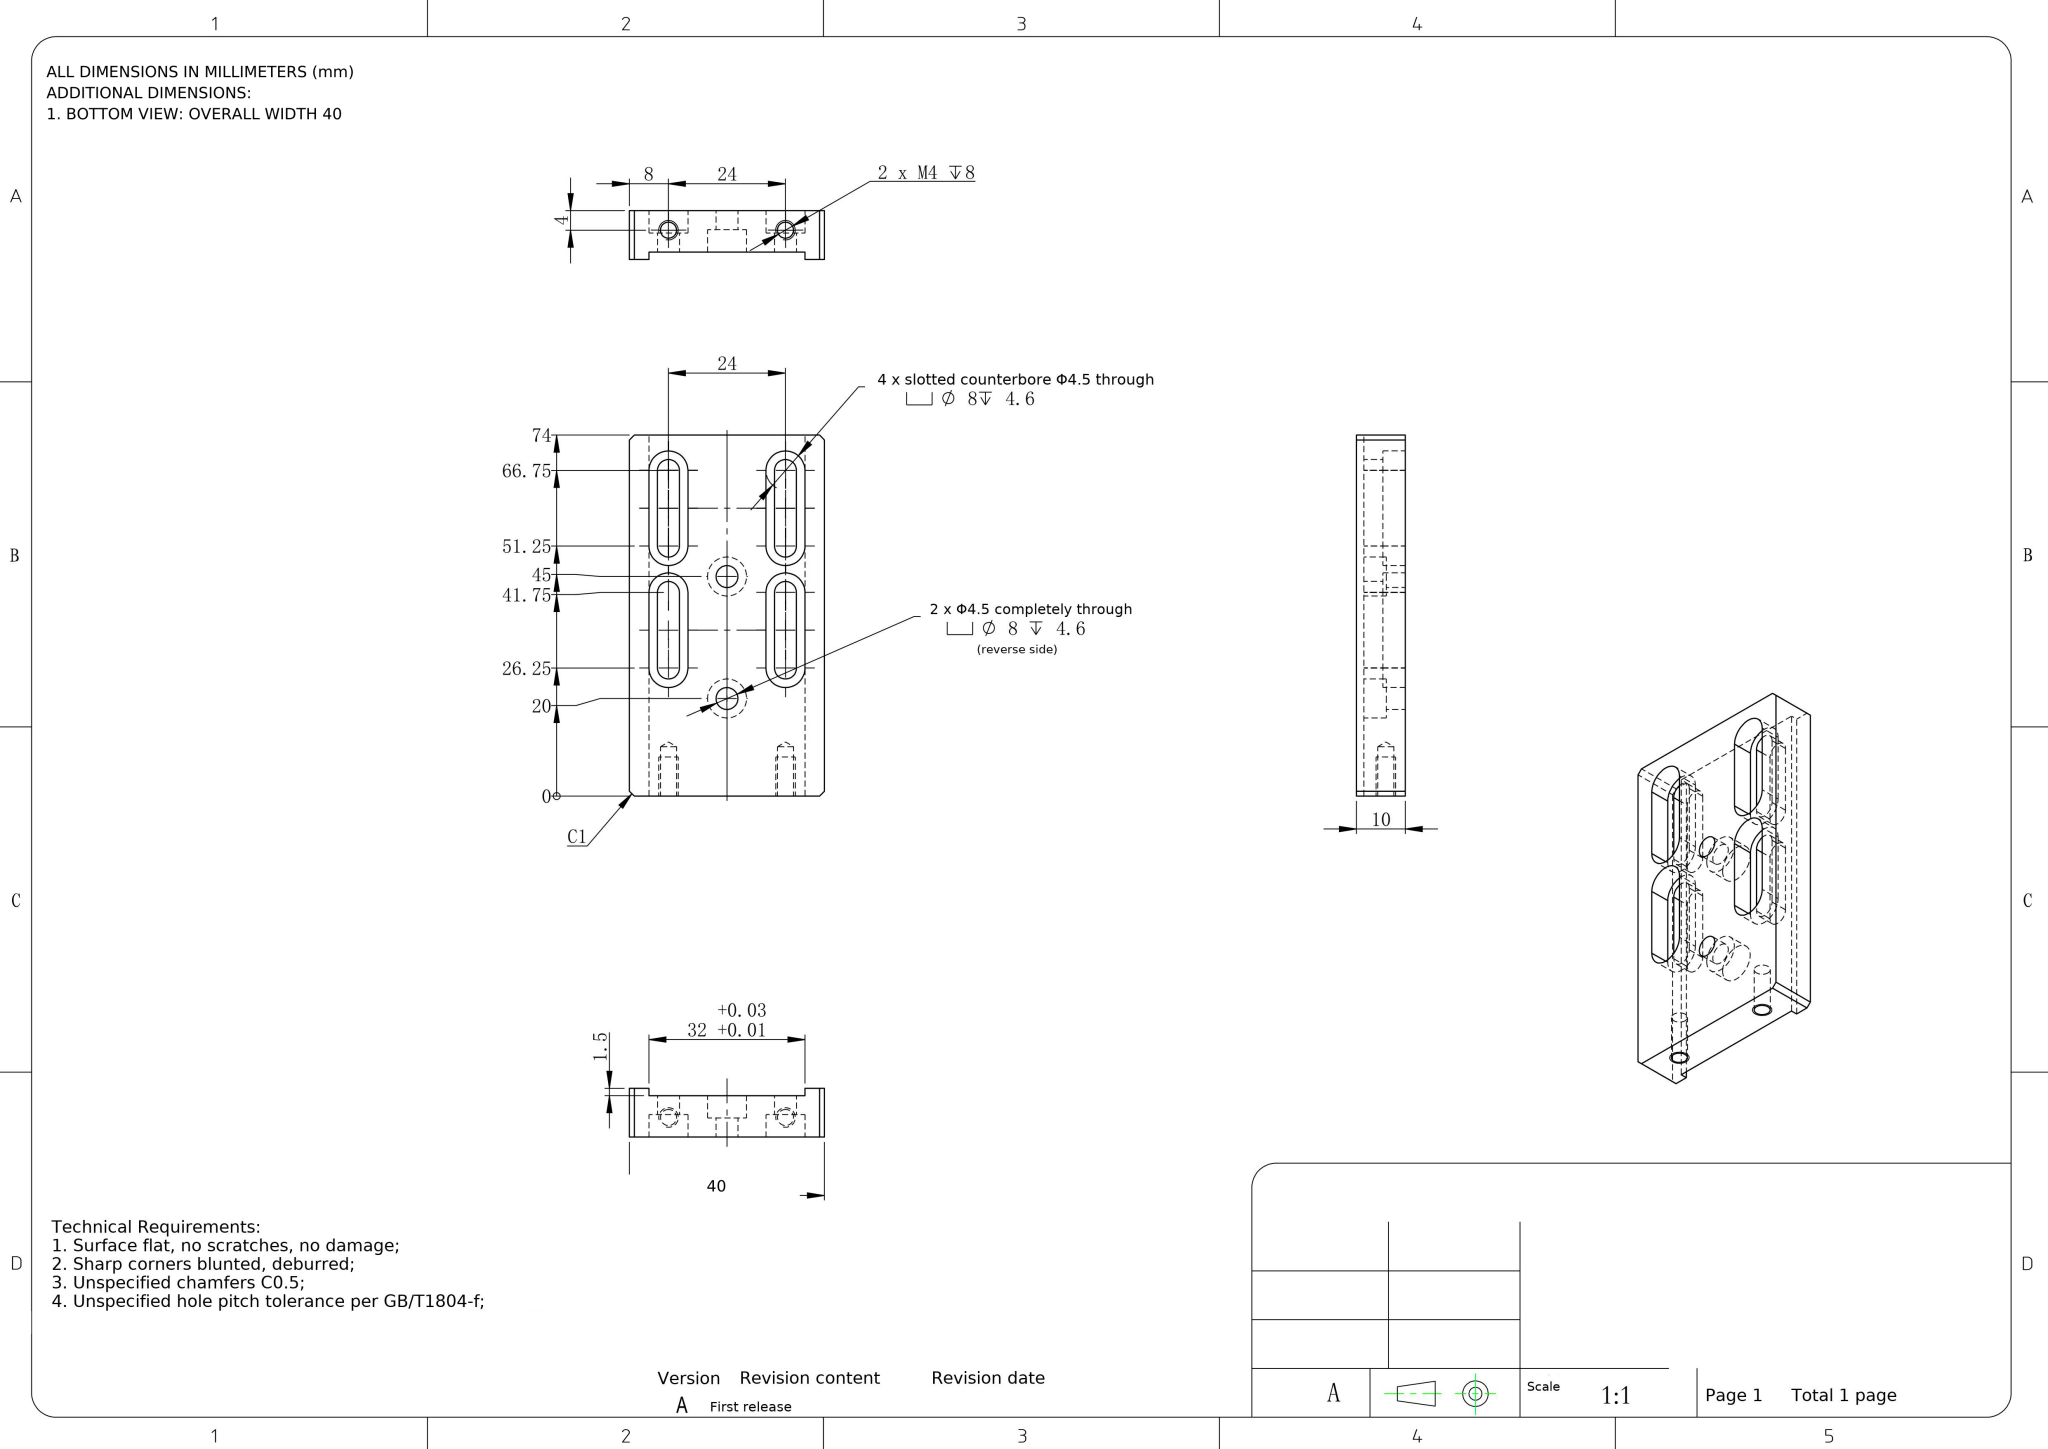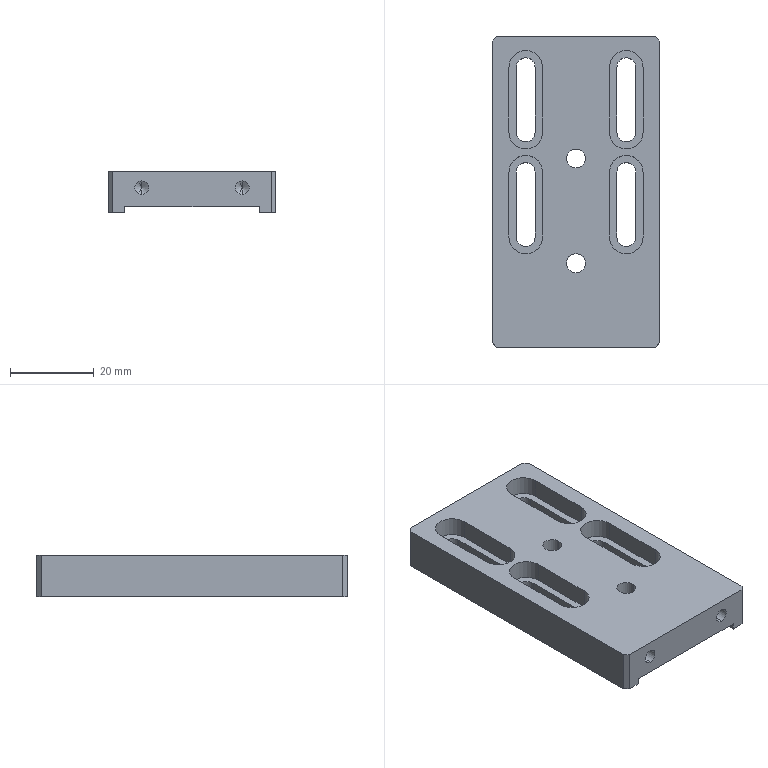Part | NX | mm | 1 solid | 68 faces | box 40 x 74 x 10 mm | volume 20720 mm3 | plane 36 | cylinder 28 | cone 4 | commonest cylinder face diameters 8 x12 4.5 x12 3.3 x4